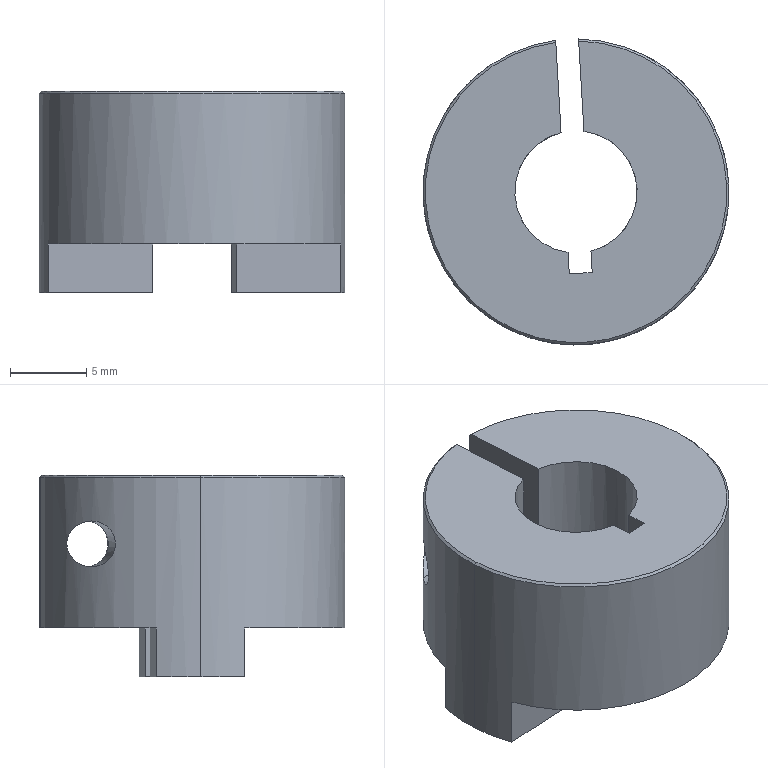Component | SolidWorks | MotorAssemblyWhen2-1_MCOCG20-8-10-1_MCOCG20-8_co2-2 | 1 solid | 32 faces | volume 2610 mm3 | plane 16 | cylinder 13 | cone 3 | commonest cylinder face diameters 20 x3 8 x3 5.6 x3 3.4 x2 3 x2